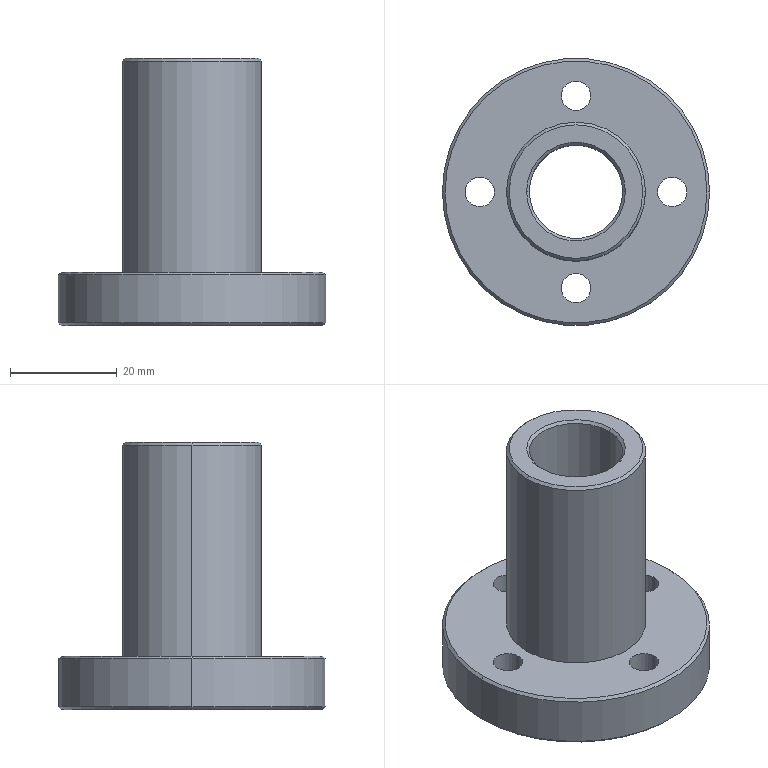Component | SolidWorks | OPW-05-011-1 | 1 solid | 39 faces | box 50 x 50 x 50 mm | volume 26737 mm3 | cylinder 22 | cone 10 | plane 7 | commonest cylinder face diameters 10 x8 5.5 x8 17.5 x2 26 x2 50 x2 | material Brass
STEP:
#1=CARTESIAN_POINT('',(-0.9411,0.4724,-1.575));
#2=VERTEX_POINT('',#1);
#3=CARTESIAN_POINT('',(0.988,0.4724,-1.575));
#4=VERTEX_POINT('',#3);
#5=CARTESIAN_POINT('',(0.02348,0.4724,-1.575));
#6=DIRECTION('',(-0.,-0.,-1.));
#7=DIRECTION('',(-1.,-0.,0.));
#8=AXIS2_PLACEMENT_3D('',#5,#6,#7);
#9=CIRCLE('',#8,0.9646);
#10=EDGE_CURVE('',#2,#4,#9,.T.);
#11=ORIENTED_EDGE('',*,*,#10,.F.);
#12=CARTESIAN_POINT('',(-0.9608,0.4724,-1.555));
#13=VERTEX_POINT('',#12);
#14=CARTESIAN_POINT('',(-0.9411,0.4724,-1.575));
#15=DIRECTION('',(-0.7071,0.,0.7071));
#16=VECTOR('',#15,39.37);
#17=LINE('',#14,#16);
#18=EDGE_CURVE('',#2,#13,#17,.T.);
#19=ORIENTED_EDGE('',*,*,#18,.T.);
#20=CARTESIAN_POINT('',(1.008,0.4724,-1.555));
#21=VERTEX_POINT('',#20);
#22=CARTESIAN_POINT('',(0.02348,0.4724,-1.555));
#23=DIRECTION('',(0.,0.,1.));
#24=DIRECTION('',(-1.,-0.,0.));
#25=AXIS2_PLACEMENT_3D('',#22,#23,#24);
#26=CIRCLE('',#25,0.9843);
#27=EDGE_CURVE('',#21,#13,#26,.T.);
#28=ORIENTED_EDGE('',*,*,#27,.F.);
#29=CARTESIAN_POINT('',(0.988,0.4724,-1.575));
#30=DIRECTION('',(0.7071,0.,0.7071));
#31=VECTOR('',#30,39.37);
#32=LINE('',#29,#31);
#33=EDGE_CURVE('',#4,#21,#32,.T.);
#34=ORIENTED_EDGE('',*,*,#33,.F.);
#35=EDGE_LOOP('',(#11,#19,#28,#34));
#36=FACE_OUTER_BOUND('',#35,.T.);
#37=CARTESIAN_POINT('',(0.02348,0.4724,-1.575));
#38=DIRECTION('',(0.,0.,1.));
#39=DIRECTION('',(1.,0.,0.));
#40=AXIS2_PLACEMENT_3D('',#37,#38,#39);
#41=CONICAL_SURFACE('',#40,0.9646,0.7854);
#42=ADVANCED_FACE('',(#36),#41,.T.);
#43=CARTESIAN_POINT('',(0.988,0.4724,-1.181));
#44=VERTEX_POINT('',#43);
#45=CARTESIAN_POINT('',(-0.9411,0.4724,-1.181));
#46=VERTEX_POINT('',#45);
#47=CARTESIAN_POINT('',(0.02348,0.4724,-1.181));
#48=DIRECTION('',(0.,0.,1.));
#49=DIRECTION('',(1.,0.,-0.));
#50=AXIS2_PLACEMENT_3D('',#47,#48,#49);
#51=CIRCLE('',#50,0.9646);
#52=EDGE_CURVE('',#44,#46,#51,.T.);
#53=ORIENTED_EDGE('',*,*,#52,.F.);
#54=CARTESIAN_POINT('',(1.008,0.4724,-1.201));
#55=VERTEX_POINT('',#54);
#56=CARTESIAN_POINT('',(0.988,0.4724,-1.181));
#57=DIRECTION('',(0.7071,0.,-0.7071));
#58=VECTOR('',#57,39.37);
#59=LINE('',#56,#58);
#60=EDGE_CURVE('',#44,#55,#59,.T.);
#61=ORIENTED_EDGE('',*,*,#60,.T.);
#62=CARTESIAN_POINT('',(-0.9608,0.4724,-1.201));
#63=VERTEX_POINT('',#62);
#64=CARTESIAN_POINT('',(0.02348,0.4724,-1.201));
#65=DIRECTION('',(-0.,-0.,-1.));
#66=DIRECTION('',(1.,0.,-0.));
#67=AXIS2_PLACEMENT_3D('',#64,#65,#66);
#68=CIRCLE('',#67,0.9843);
#69=EDGE_CURVE('',#63,#55,#68,.T.);
#70=ORIENTED_EDGE('',*,*,#69,.F.);
#71=CARTESIAN_POINT('',(-0.9411,0.4724,-1.181));
#72=DIRECTION('',(-0.7071,-0.,-0.7071));
#73=VECTOR('',#72,39.37);
#74=LINE('',#71,#73);
#75=EDGE_CURVE('',#46,#63,#74,.T.);
#76=ORIENTED_EDGE('',*,*,#75,.F.);
#77=EDGE_LOOP('',(#53,#61,#70,#76));
#78=FACE_OUTER_BOUND('',#77,.T.);
#79=CARTESIAN_POINT('',(0.02348,0.4724,-1.181));
#80=DIRECTION('',(-0.,-0.,-1.));
#81=DIRECTION('',(-1.,-0.,0.));
#82=AXIS2_PLACEMENT_3D('',#79,#80,#81);
#83=CONICAL_SURFACE('',#82,0.9646,0.7854);
#84=ADVANCED_FACE('',(#78),#83,.T.);
#85=CARTESIAN_POINT('',(0.368,0.4724,-1.555));
#86=VERTEX_POINT('',#85);
#87=CARTESIAN_POINT('',(-0.321,0.4724,-1.555));
#88=VERTEX_POINT('',#87);
#89=CARTESIAN_POINT('',(0.02348,0.4724,-1.555));
#90=DIRECTION('',(-0.,-0.,-1.));
#91=DIRECTION('',(-1.,0.,0.));
#92=AXIS2_PLACEMENT_3D('',#89,#90,#91);
#93=CIRCLE('',#92,0.3445);
#94=EDGE_CURVE('',#86,#88,#93,.T.);
#95=ORIENTED_EDGE('',*,*,#94,.F.);
#96=CARTESIAN_POINT('',(0.3877,0.4724,-1.575));
#97=VERTEX_POINT('',#96);
#98=CARTESIAN_POINT('',(0.368,0.4724,-1.555));
#99=DIRECTION('',(0.7071,0.,-0.7071));
#100=VECTOR('',#99,39.37);
#101=LINE('',#98,#100);
#102=EDGE_CURVE('',#86,#97,#101,.T.);
#103=ORIENTED_EDGE('',*,*,#102,.T.);
#104=CARTESIAN_POINT('',(-0.3407,0.4724,-1.575));
#105=VERTEX_POINT('',#104);
#106=CARTESIAN_POINT('',(0.02348,0.4724,-1.575));
#107=DIRECTION('',(0.,0.,1.));
#108=DIRECTION('',(-1.,0.,0.));
#109=AXIS2_PLACEMENT_3D('',#106,#107,#108);
#110=CIRCLE('',#109,0.3642);
#111=EDGE_CURVE('',#105,#97,#110,.T.);
#112=ORIENTED_EDGE('',*,*,#111,.F.);
#113=CARTESIAN_POINT('',(-0.321,0.4724,-1.555));
#114=DIRECTION('',(-0.7071,-0.,-0.7071));
#115=VECTOR('',#114,39.37);
#116=LINE('',#113,#115);
#117=EDGE_CURVE('',#88,#105,#116,.T.);
#118=ORIENTED_EDGE('',*,*,#117,.F.);
#119=EDGE_LOOP('',(#95,#103,#112,#118));
#120=FACE_OUTER_BOUND('',#119,.T.);
#121=CARTESIAN_POINT('',(0.02348,0.4724,-1.555));
#122=DIRECTION('',(-0.,-0.,-1.));
#123=DIRECTION('',(-1.,0.,0.));
#124=AXIS2_PLACEMENT_3D('',#121,#122,#123);
#125=CONICAL_SURFACE('',#124,0.3445,0.7854);
#126=ADVANCED_FACE('',(#120),#125,.F.);
#127=CARTESIAN_POINT('',(-0.321,0.4724,0.374));
#128=VERTEX_POINT('',#127);
#129=CARTESIAN_POINT('',(0.368,0.4724,0.374));
#130=VERTEX_POINT('',#129);
#131=CARTESIAN_POINT('',(0.02348,0.4724,0.374));
#132=DIRECTION('',(0.,0.,1.));
#133=DIRECTION('',(-1.,0.,0.));
#134=AXIS2_PLACEMENT_3D('',#131,#132,#133);
#135=CIRCLE('',#134,0.3445);
#136=EDGE_CURVE('',#128,#130,#135,.T.);
#137=ORIENTED_EDGE('',*,*,#136,.F.);
#138=CARTESIAN_POINT('',(-0.3407,0.4724,0.3937));
#139=VERTEX_POINT('',#138);
#140=CARTESIAN_POINT('',(-0.3407,0.4724,0.3937));
#141=DIRECTION('',(-0.7071,0.,0.7071));
#142=VECTOR('',#141,39.37);
#143=LINE('',#140,#142);
#144=EDGE_CURVE('',#128,#139,#143,.T.);
#145=ORIENTED_EDGE('',*,*,#144,.T.);
#146=CARTESIAN_POINT('',(0.3877,0.4724,0.3937));
#147=VERTEX_POINT('',#146);
#148=CARTESIAN_POINT('',(0.02348,0.4724,0.3937));
#149=DIRECTION('',(-0.,-0.,-1.));
#150=DIRECTION('',(-1.,0.,0.));
#151=AXIS2_PLACEMENT_3D('',#148,#149,#150);
#152=CIRCLE('',#151,0.3642);
#153=EDGE_CURVE('',#147,#139,#152,.T.);
#154=ORIENTED_EDGE('',*,*,#153,.F.);
#155=CARTESIAN_POINT('',(0.3877,0.4724,0.3937));
#156=DIRECTION('',(0.7071,0.,0.7071));
#157=VECTOR('',#156,39.37);
#158=LINE('',#155,#157);
#159=EDGE_CURVE('',#130,#147,#158,.T.);
#160=ORIENTED_EDGE('',*,*,#159,.F.);
#161=EDGE_LOOP('',(#137,#145,#154,#160));
#162=FACE_OUTER_BOUND('',#161,.T.);
#163=CARTESIAN_POINT('',(0.02348,0.4724,0.3937));
#164=DIRECTION('',(0.,0.,1.));
#165=DIRECTION('',(1.,0.,-0.));
#166=AXIS2_PLACEMENT_3D('',#163,#164,#165);
#167=CONICAL_SURFACE('',#166,0.3642,0.7854);
#168=ADVANCED_FACE('',(#162),#167,.F.);
#169=CARTESIAN_POINT('',(0.5156,0.4724,0.3937));
#170=VERTEX_POINT('',#169);
#171=CARTESIAN_POINT('',(-0.4686,0.4724,0.3937));
#172=VERTEX_POINT('',#171);
#173=CARTESIAN_POINT('',(0.02348,0.4724,0.3937));
#174=DIRECTION('',(0.,0.,1.));
#175=DIRECTION('',(-1.,0.,0.));
#176=AXIS2_PLACEMENT_3D('',#173,#174,#175);
#177=CIRCLE('',#176,0.4921);
#178=EDGE_CURVE('',#170,#172,#177,.T.);
#179=ORIENTED_EDGE('',*,*,#178,.F.);
#180=CARTESIAN_POINT('',(0.5353,0.4724,0.374));
#181=VERTEX_POINT('',#180);
#182=CARTESIAN_POINT('',(0.5156,0.4724,0.3937));
#183=DIRECTION('',(0.7071,0.,-0.7071));
#184=VECTOR('',#183,39.37);
#185=LINE('',#182,#184);
#186=EDGE_CURVE('',#170,#181,#185,.T.);
#187=ORIENTED_EDGE('',*,*,#186,.T.);
#188=CARTESIAN_POINT('',(-0.4883,0.4724,0.374));
#189=VERTEX_POINT('',#188);
#190=CARTESIAN_POINT('',(0.02348,0.4724,0.374));
#191=DIRECTION('',(-0.,-0.,-1.));
#192=DIRECTION('',(-1.,0.,0.));
#193=AXIS2_PLACEMENT_3D('',#190,#191,#192);
#194=CIRCLE('',#193,0.5118);
#195=EDGE_CURVE('',#189,#181,#194,.T.);
#196=ORIENTED_EDGE('',*,*,#195,.F.);
#197=CARTESIAN_POINT('',(-0.4686,0.4724,0.3937));
#198=DIRECTION('',(-0.7071,-0.,-0.7071));
#199=VECTOR('',#198,39.37);
#200=LINE('',#197,#199);
#201=EDGE_CURVE('',#172,#189,#200,.T.);
#202=ORIENTED_EDGE('',*,*,#201,.F.);
#203=EDGE_LOOP('',(#179,#187,#196,#202));
#204=FACE_OUTER_BOUND('',#203,.T.);
#205=CARTESIAN_POINT('',(0.02348,0.4724,0.3937));
#206=DIRECTION('',(-0.,-0.,-1.));
#207=DIRECTION('',(-1.,0.,0.));
#208=AXIS2_PLACEMENT_3D('',#205,#206,#207);
#209=CONICAL_SURFACE('',#208,0.4921,0.7854);
#210=ADVANCED_FACE('',(#204),#209,.T.);
#211=CARTESIAN_POINT('',(0.929,0.4724,-1.378));
#212=VERTEX_POINT('',#211);
#213=CARTESIAN_POINT('',(0.5353,0.4724,-1.378));
#214=VERTEX_POINT('',#213);
#215=CARTESIAN_POINT('',(0.7321,0.4724,-1.378));
#216=DIRECTION('',(-0.,-0.,-1.));
#217=DIRECTION('',(-1.,0.,0.));
#218=AXIS2_PLACEMENT_3D('',#215,#216,#217);
#219=CIRCLE('',#218,0.1969);
#220=EDGE_CURVE('',#212,#214,#219,.T.);
#221=ORIENTED_EDGE('',*,*,#220,.F.);
#222=CARTESIAN_POINT('',(0.929,0.4724,-1.575));
#223=VERTEX_POINT('',#222);
#224=CARTESIAN_POINT('',(0.929,0.4724,-1.575));
#225=DIRECTION('',(-0.,-0.,-1.));
#226=VECTOR('',#225,39.37);
#227=LINE('',#224,#226);
#228=EDGE_CURVE('',#212,#223,#227,.T.);
#229=ORIENTED_EDGE('',*,*,#228,.T.);
#230=CARTESIAN_POINT('',(0.5353,0.4724,-1.575));
#231=VERTEX_POINT('',#230);
#232=CARTESIAN_POINT('',(0.7321,0.4724,-1.575));
#233=DIRECTION('',(-0.,-0.,-1.));
#234=DIRECTION('',(-1.,0.,0.));
#235=AXIS2_PLACEMENT_3D('',#232,#233,#234);
#236=CIRCLE('',#235,0.1969);
#237=EDGE_CURVE('',#223,#231,#236,.T.);
#238=ORIENTED_EDGE('',*,*,#237,.T.);
#239=CARTESIAN_POINT('',(0.5353,0.4724,-1.575));
#240=DIRECTION('',(-0.,-0.,-1.));
#241=VECTOR('',#240,39.37);
#242=LINE('',#239,#241);
#243=EDGE_CURVE('',#214,#231,#242,.T.);
#244=ORIENTED_EDGE('',*,*,#243,.F.);
#245=EDGE_LOOP('',(#221,#229,#238,#244));
#246=FACE_OUTER_BOUND('',#245,.T.);
#247=CARTESIAN_POINT('',(0.7321,0.4724,-1.575));
#248=DIRECTION('',(-0.,-0.,-1.));
#249=DIRECTION('',(-1.,0.,0.));
#250=AXIS2_PLACEMENT_3D('',#247,#248,#249);
#251=CYLINDRICAL_SURFACE('',#250,0.1969);
#252=ADVANCED_FACE('',(#246),#251,.F.);
#253=CARTESIAN_POINT('',(0.6239,0.4724,-1.181));
#254=VERTEX_POINT('',#253);
#255=CARTESIAN_POINT('',(0.8404,0.4724,-1.181));
#256=VERTEX_POINT('',#255);
#257=CARTESIAN_POINT('',(0.7321,0.4724,-1.181));
#258=DIRECTION('',(0.,0.,1.));
#259=DIRECTION('',(1.,0.,0.));
#260=AXIS2_PLACEMENT_3D('',#257,#258,#259);
#261=CIRCLE('',#260,0.1083);
#262=EDGE_CURVE('',#254,#256,#261,.T.);
#263=ORIENTED_EDGE('',*,*,#262,.T.);
#264=CARTESIAN_POINT('',(0.8404,0.4724,-1.378));
#265=VERTEX_POINT('',#264);
#266=CARTESIAN_POINT('',(0.8404,0.4724,-1.575));
#267=DIRECTION('',(-0.,-0.,-1.));
#268=VECTOR('',#267,39.37);
#269=LINE('',#266,#268);
#270=EDGE_CURVE('',#256,#265,#269,.T.);
#271=ORIENTED_EDGE('',*,*,#270,.T.);
#272=CARTESIAN_POINT('',(0.6239,0.4724,-1.378));
#273=VERTEX_POINT('',#272);
#274=CARTESIAN_POINT('',(0.7321,0.4724,-1.378));
#275=DIRECTION('',(-0.,-0.,-1.));
#276=DIRECTION('',(-1.,0.,0.));
#277=AXIS2_PLACEMENT_3D('',#274,#275,#276);
#278=CIRCLE('',#277,0.1083);
#279=EDGE_CURVE('',#265,#273,#278,.T.);
#280=ORIENTED_EDGE('',*,*,#279,.T.);
#281=CARTESIAN_POINT('',(0.6239,0.4724,-1.575));
#282=DIRECTION('',(-0.,-0.,-1.));
#283=VECTOR('',#282,39.37);
#284=LINE('',#281,#283);
#285=EDGE_CURVE('',#254,#273,#284,.T.);
#286=ORIENTED_EDGE('',*,*,#285,.F.);
#287=EDGE_LOOP('',(#263,#271,#280,#286));
#288=FACE_OUTER_BOUND('',#287,.T.);
#289=CARTESIAN_POINT('',(0.7321,0.4724,-1.575));
#290=DIRECTION('',(-0.,-0.,-1.));
#291=DIRECTION('',(-1.,0.,0.));
#292=AXIS2_PLACEMENT_3D('',#289,#290,#291);
#293=CYLINDRICAL_SURFACE('',#292,0.1083);
#294=ADVANCED_FACE('',(#288),#293,.F.);
#295=CARTESIAN_POINT('',(0.2203,-0.2363,-1.378));
#296=VERTEX_POINT('',#295);
#297=CARTESIAN_POINT('',(-0.1734,-0.2363,-1.378));
#298=VERTEX_POINT('',#297);
#299=CARTESIAN_POINT('',(0.02348,-0.2363,-1.378));
#300=DIRECTION('',(-0.,-0.,-1.));
#301=DIRECTION('',(-1.,0.,0.));
#302=AXIS2_PLACEMENT_3D('',#299,#300,#301);
#303=CIRCLE('',#302,0.1969);
#304=EDGE_CURVE('',#296,#298,#303,.T.);
#305=ORIENTED_EDGE('',*,*,#304,.F.);
#306=CARTESIAN_POINT('',(0.2203,-0.2363,-1.575));
#307=VERTEX_POINT('',#306);
#308=CARTESIAN_POINT('',(0.2203,-0.2363,-1.575));
#309=DIRECTION('',(-0.,-0.,-1.));
#310=VECTOR('',#309,39.37);
#311=LINE('',#308,#310);
#312=EDGE_CURVE('',#296,#307,#311,.T.);
#313=ORIENTED_EDGE('',*,*,#312,.T.);
#314=CARTESIAN_POINT('',(-0.1734,-0.2363,-1.575));
#315=VERTEX_POINT('',#314);
#316=CARTESIAN_POINT('',(0.02348,-0.2363,-1.575));
#317=DIRECTION('',(-0.,-0.,-1.));
#318=DIRECTION('',(-1.,0.,0.));
#319=AXIS2_PLACEMENT_3D('',#316,#317,#318);
#320=CIRCLE('',#319,0.1969);
#321=EDGE_CURVE('',#307,#315,#320,.T.);
#322=ORIENTED_EDGE('',*,*,#321,.T.);
#323=CARTESIAN_POINT('',(-0.1734,-0.2363,-1.575));
#324=DIRECTION('',(-0.,-0.,-1.));
#325=VECTOR('',#324,39.37);
#326=LINE('',#323,#325);
#327=EDGE_CURVE('',#298,#315,#326,.T.);
#328=ORIENTED_EDGE('',*,*,#327,.F.);
#329=EDGE_LOOP('',(#305,#313,#322,#328));
#330=FACE_OUTER_BOUND('',#329,.T.);
#331=CARTESIAN_POINT('',(0.02348,-0.2363,-1.575));
#332=DIRECTION('',(-0.,-0.,-1.));
#333=DIRECTION('',(-1.,0.,0.));
#334=AXIS2_PLACEMENT_3D('',#331,#332,#333);
#335=CYLINDRICAL_SURFACE('',#334,0.1969);
#336=ADVANCED_FACE('',(#330),#335,.F.);
#337=CARTESIAN_POINT('',(-0.08478,-0.2363,-1.181));
#338=VERTEX_POINT('',#337);
#339=CARTESIAN_POINT('',(0.1318,-0.2363,-1.181));
#340=VERTEX_POINT('',#339);
#341=CARTESIAN_POINT('',(0.02348,-0.2363,-1.181));
#342=DIRECTION('',(0.,0.,1.));
#343=DIRECTION('',(1.,0.,0.));
#344=AXIS2_PLACEMENT_3D('',#341,#342,#343);
#345=CIRCLE('',#344,0.1083);
#346=EDGE_CURVE('',#338,#340,#345,.T.);
#347=ORIENTED_EDGE('',*,*,#346,.T.);
#348=CARTESIAN_POINT('',(0.1318,-0.2363,-1.378));
#349=VERTEX_POINT('',#348);
#350=CARTESIAN_POINT('',(0.1318,-0.2363,-1.575));
#351=DIRECTION('',(-0.,-0.,-1.));
#352=VECTOR('',#351,39.37);
#353=LINE('',#350,#352);
#354=EDGE_CURVE('',#340,#349,#353,.T.);
#355=ORIENTED_EDGE('',*,*,#354,.T.);
#356=CARTESIAN_POINT('',(-0.08478,-0.2363,-1.378));
#357=VERTEX_POINT('',#356);
#358=CARTESIAN_POINT('',(0.02348,-0.2363,-1.378));
#359=DIRECTION('',(-0.,-0.,-1.));
#360=DIRECTION('',(-1.,0.,0.));
#361=AXIS2_PLACEMENT_3D('',#358,#359,#360);
#362=CIRCLE('',#361,0.1083);
#363=EDGE_CURVE('',#349,#357,#362,.T.);
#364=ORIENTED_EDGE('',*,*,#363,.T.);
#365=CARTESIAN_POINT('',(-0.08478,-0.2363,-1.575));
#366=DIRECTION('',(-0.,-0.,-1.));
#367=VECTOR('',#366,39.37);
#368=LINE('',#365,#367);
#369=EDGE_CURVE('',#338,#357,#368,.T.);
#370=ORIENTED_EDGE('',*,*,#369,.F.);
#371=EDGE_LOOP('',(#347,#355,#364,#370));
#372=FACE_OUTER_BOUND('',#371,.T.);
#373=CARTESIAN_POINT('',(0.02348,-0.2363,-1.575));
#374=DIRECTION('',(-0.,-0.,-1.));
#375=DIRECTION('',(-1.,0.,0.));
#376=AXIS2_PLACEMENT_3D('',#373,#374,#375);
#377=CYLINDRICAL_SURFACE('',#376,0.1083);
#378=ADVANCED_FACE('',(#372),#377,.F.);
#379=CARTESIAN_POINT('',(-0.4883,0.4724,-1.378));
#380=VERTEX_POINT('',#379);
#381=CARTESIAN_POINT('',(-0.882,0.4724,-1.378));
#382=VERTEX_POINT('',#381);
#383=CARTESIAN_POINT('',(-0.6852,0.4724,-1.378));
#384=DIRECTION('',(-0.,-0.,-1.));
#385=DIRECTION('',(-1.,0.,0.));
#386=AXIS2_PLACEMENT_3D('',#383,#384,#385);
#387=CIRCLE('',#386,0.1969);
#388=EDGE_CURVE('',#380,#382,#387,.T.);
#389=ORIENTED_EDGE('',*,*,#388,.F.);
#390=CARTESIAN_POINT('',(-0.4883,0.4724,-1.575));
#391=VERTEX_POINT('',#390);
#392=CARTESIAN_POINT('',(-0.4883,0.4724,-1.575));
#393=DIRECTION('',(-0.,-0.,-1.));
#394=VECTOR('',#393,39.37);
#395=LINE('',#392,#394);
#396=EDGE_CURVE('',#380,#391,#395,.T.);
#397=ORIENTED_EDGE('',*,*,#396,.T.);
#398=CARTESIAN_POINT('',(-0.882,0.4724,-1.575));
#399=VERTEX_POINT('',#398);
#400=CARTESIAN_POINT('',(-0.6852,0.4724,-1.575));
#401=DIRECTION('',(-0.,-0.,-1.));
#402=DIRECTION('',(-1.,0.,0.));
#403=AXIS2_PLACEMENT_3D('',#400,#401,#402);
#404=CIRCLE('',#403,0.1969);
#405=EDGE_CURVE('',#391,#399,#404,.T.);
#406=ORIENTED_EDGE('',*,*,#405,.T.);
#407=CARTESIAN_POINT('',(-0.882,0.4724,-1.575));
#408=DIRECTION('',(-0.,-0.,-1.));
#409=VECTOR('',#408,39.37);
#410=LINE('',#407,#409);
#411=EDGE_CURVE('',#382,#399,#410,.T.);
#412=ORIENTED_EDGE('',*,*,#411,.F.);
#413=EDGE_LOOP('',(#389,#397,#406,#412));
#414=FACE_OUTER_BOUND('',#413,.T.);
#415=CARTESIAN_POINT('',(-0.6852,0.4724,-1.575));
#416=DIRECTION('',(-0.,-0.,-1.));
#417=DIRECTION('',(-1.,0.,0.));
#418=AXIS2_PLACEMENT_3D('',#415,#416,#417);
#419=CYLINDRICAL_SURFACE('',#418,0.1969);
#420=ADVANCED_FACE('',(#414),#419,.F.);
#421=CARTESIAN_POINT('',(-0.7934,0.4724,-1.181));
#422=VERTEX_POINT('',#421);
#423=CARTESIAN_POINT('',(-0.5769,0.4724,-1.181));
#424=VERTEX_POINT('',#423);
#425=CARTESIAN_POINT('',(-0.6852,0.4724,-1.181));
#426=DIRECTION('',(0.,0.,1.));
#427=DIRECTION('',(1.,0.,0.));
#428=AXIS2_PLACEMENT_3D('',#425,#426,#427);
#429=CIRCLE('',#428,0.1083);
#430=EDGE_CURVE('',#422,#424,#429,.T.);
#431=ORIENTED_EDGE('',*,*,#430,.T.);
#432=CARTESIAN_POINT('',(-0.5769,0.4724,-1.378));
#433=VERTEX_POINT('',#432);
#434=CARTESIAN_POINT('',(-0.5769,0.4724,-1.575));
#435=DIRECTION('',(-0.,-0.,-1.));
#436=VECTOR('',#435,39.37);
#437=LINE('',#434,#436);
#438=EDGE_CURVE('',#424,#433,#437,.T.);
#439=ORIENTED_EDGE('',*,*,#438,.T.);
#440=CARTESIAN_POINT('',(-0.7934,0.4724,-1.378));
#441=VERTEX_POINT('',#440);
#442=CARTESIAN_POINT('',(-0.6852,0.4724,-1.378));
#443=DIRECTION('',(-0.,-0.,-1.));
#444=DIRECTION('',(-1.,0.,0.));
#445=AXIS2_PLACEMENT_3D('',#442,#443,#444);
#446=CIRCLE('',#445,0.1083);
#447=EDGE_CURVE('',#433,#441,#446,.T.);
#448=ORIENTED_EDGE('',*,*,#447,.T.);
#449=CARTESIAN_POINT('',(-0.7934,0.4724,-1.575));
#450=DIRECTION('',(-0.,-0.,-1.));
#451=VECTOR('',#450,39.37);
#452=LINE('',#449,#451);
#453=EDGE_CURVE('',#422,#441,#452,.T.);
#454=ORIENTED_EDGE('',*,*,#453,.F.);
#455=EDGE_LOOP('',(#431,#439,#448,#454));
#456=FACE_OUTER_BOUND('',#455,.T.);
#457=CARTESIAN_POINT('',(-0.6852,0.4724,-1.575));
#458=DIRECTION('',(-0.,-0.,-1.));
#459=DIRECTION('',(-1.,0.,0.));
#460=AXIS2_PLACEMENT_3D('',#457,#458,#459);
#461=CYLINDRICAL_SURFACE('',#460,0.1083);
#462=ADVANCED_FACE('',(#456),#461,.F.);
#463=CARTESIAN_POINT('',(0.2203,1.181,-1.378));
#464=VERTEX_POINT('',#463);
#465=CARTESIAN_POINT('',(-0.1734,1.181,-1.378));
#466=VERTEX_POINT('',#465);
#467=CARTESIAN_POINT('',(0.02348,1.181,-1.378));
#468=DIRECTION('',(-0.,-0.,-1.));
#469=DIRECTION('',(-1.,0.,0.));
#470=AXIS2_PLACEMENT_3D('',#467,#468,#469);
#471=CIRCLE('',#470,0.1969);
#472=EDGE_CURVE('',#464,#466,#471,.T.);
#473=ORIENTED_EDGE('',*,*,#472,.F.);
#474=CARTESIAN_POINT('',(0.2203,1.181,-1.575));
#475=VERTEX_POINT('',#474);
#476=CARTESIAN_POINT('',(0.2203,1.181,-1.575));
#477=DIRECTION('',(-0.,-0.,-1.));
#478=VECTOR('',#477,39.37);
#479=LINE('',#476,#478);
#480=EDGE_CURVE('',#464,#475,#479,.T.);
#481=ORIENTED_EDGE('',*,*,#480,.T.);
#482=CARTESIAN_POINT('',(-0.1734,1.181,-1.575));
#483=VERTEX_POINT('',#482);
#484=CARTESIAN_POINT('',(0.02348,1.181,-1.575));
#485=DIRECTION('',(-0.,-0.,-1.));
#486=DIRECTION('',(-1.,0.,0.));
#487=AXIS2_PLACEMENT_3D('',#484,#485,#486);
#488=CIRCLE('',#487,0.1969);
#489=EDGE_CURVE('',#475,#483,#488,.T.);
#490=ORIENTED_EDGE('',*,*,#489,.T.);
#491=CARTESIAN_POINT('',(-0.1734,1.181,-1.575));
#492=DIRECTION('',(-0.,-0.,-1.));
#493=VECTOR('',#492,39.37);
#494=LINE('',#491,#493);
#495=EDGE_CURVE('',#466,#483,#494,.T.);
#496=ORIENTED_EDGE('',*,*,#495,.F.);
#497=EDGE_LOOP('',(#473,#481,#490,#496));
#498=FACE_OUTER_BOUND('',#497,.T.);
#499=CARTESIAN_POINT('',(0.02348,1.181,-1.575));
#500=DIRECTION('',(-0.,-0.,-1.));
#501=DIRECTION('',(-1.,0.,0.));
#502=AXIS2_PLACEMENT_3D('',#499,#500,#501);
#503=CYLINDRICAL_SURFACE('',#502,0.1969);
#504=ADVANCED_FACE('',(#498),#503,.F.);
#505=CARTESIAN_POINT('',(-0.08478,1.181,-1.181));
#506=VERTEX_POINT('',#505);
#507=CARTESIAN_POINT('',(0.1318,1.181,-1.181));
#508=VERTEX_POINT('',#507);
#509=CARTESIAN_POINT('',(0.02348,1.181,-1.181));
#510=DIRECTION('',(0.,0.,1.));
#511=DIRECTION('',(1.,0.,0.));
#512=AXIS2_PLACEMENT_3D('',#509,#510,#511);
#513=CIRCLE('',#512,0.1083);
#514=EDGE_CURVE('',#506,#508,#513,.T.);
#515=ORIENTED_EDGE('',*,*,#514,.T.);
#516=CARTESIAN_POINT('',(0.1318,1.181,-1.378));
#517=VERTEX_POINT('',#516);
#518=CARTESIAN_POINT('',(0.1318,1.181,-1.575));
#519=DIRECTION('',(-0.,-0.,-1.));
#520=VECTOR('',#519,39.37);
#521=LINE('',#518,#520);
#522=EDGE_CURVE('',#508,#517,#521,.T.);
#523=ORIENTED_EDGE('',*,*,#522,.T.);
#524=CARTESIAN_POINT('',(-0.08478,1.181,-1.378));
#525=VERTEX_POINT('',#524);
#526=CARTESIAN_POINT('',(0.02348,1.181,-1.378));
#527=DIRECTION('',(-0.,-0.,-1.));
#528=DIRECTION('',(-1.,0.,0.));
#529=AXIS2_PLACEMENT_3D('',#526,#527,#528);
#530=CIRCLE('',#529,0.1083);
#531=EDGE_CURVE('',#517,#525,#530,.T.);
#532=ORIENTED_EDGE('',*,*,#531,.T.);
#533=CARTESIAN_POINT('',(-0.08478,1.181,-1.575));
#534=DIRECTION('',(-0.,-0.,-1.));
#535=VECTOR('',#534,39.37);
#536=LINE('',#533,#535);
#537=EDGE_CURVE('',#506,#525,#536,.T.);
#538=ORIENTED_EDGE('',*,*,#537,.F.);
#539=EDGE_LOOP('',(#515,#523,#532,#538));
#540=FACE_OUTER_BOUND('',#539,.T.);
#541=CARTESIAN_POINT('',(0.02348,1.181,-1.575));
#542=DIRECTION('',(-0.,-0.,-1.));
#543=DIRECTION('',(-1.,0.,0.));
#544=AXIS2_PLACEMENT_3D('',#541,#542,#543);
#545=CYLINDRICAL_SURFACE('',#544,0.1083);
#546=ADVANCED_FACE('',(#540),#545,.F.);
#547=ORIENTED_EDGE('',*,*,#136,.T.);
#548=CARTESIAN_POINT('',(0.368,0.4724,-1.575));
#549=DIRECTION('',(-0.,-0.,-1.));
#550=VECTOR('',#549,39.37);
#551=LINE('',#548,#550);
#552=EDGE_CURVE('',#130,#86,#551,.T.);
#553=ORIENTED_EDGE('',*,*,#552,.T.);
#554=ORIENTED_EDGE('',*,*,#94,.T.);
#555=CARTESIAN_POINT('',(-0.321,0.4724,-1.575));
#556=DIRECTION('',(-0.,-0.,-1.));
#557=VECTOR('',#556,39.37);
#558=LINE('',#555,#557);
#559=EDGE_CURVE('',#128,#88,#558,.T.);
#560=ORIENTED_EDGE('',*,*,#559,.F.);
#561=EDGE_LOOP('',(#547,#553,#554,#560));
#562=FACE_OUTER_BOUND('',#561,.T.);
#563=CARTESIAN_POINT('',(0.02348,0.4724,-1.575));
#564=DIRECTION('',(-0.,-0.,-1.));
#565=DIRECTION('',(-1.,0.,0.));
#566=AXIS2_PLACEMENT_3D('',#563,#564,#565);
#567=CYLINDRICAL_SURFACE('',#566,0.3445);
#568=ADVANCED_FACE('',(#562),#567,.F.);
#569=CARTESIAN_POINT('',(0.5353,0.4724,-1.181));
#570=VERTEX_POINT('',#569);
#571=CARTESIAN_POINT('',(-0.4883,0.4724,-1.181));
#572=VERTEX_POINT('',#571);
#573=CARTESIAN_POINT('',(0.02348,0.4724,-1.181));
#574=DIRECTION('',(0.,0.,1.));
#575=DIRECTION('',(1.,0.,0.));
#576=AXIS2_PLACEMENT_3D('',#573,#574,#575);
#577=CIRCLE('',#576,0.5118);
#578=EDGE_CURVE('',#570,#572,#577,.T.);
#579=ORIENTED_EDGE('',*,*,#578,.T.);
#580=CARTESIAN_POINT('',(-0.4883,0.4724,-1.181));
#581=DIRECTION('',(0.,0.,1.));
#582=VECTOR('',#581,39.37);
#583=LINE('',#580,#582);
#584=EDGE_CURVE('',#572,#189,#583,.T.);
#585=ORIENTED_EDGE('',*,*,#584,.T.);
#586=ORIENTED_EDGE('',*,*,#195,.T.);
#587=CARTESIAN_POINT('',(0.5353,0.4724,-1.181));
#588=DIRECTION('',(0.,0.,1.));
#589=VECTOR('',#588,39.37);
#590=LINE('',#587,#589);
#591=EDGE_CURVE('',#570,#181,#590,.T.);
#592=ORIENTED_EDGE('',*,*,#591,.F.);
#593=EDGE_LOOP('',(#579,#585,#586,#592));
#594=FACE_OUTER_BOUND('',#593,.T.);
#595=CARTESIAN_POINT('',(0.02348,0.4724,-1.181));
#596=DIRECTION('',(0.,0.,1.));
#597=DIRECTION('',(1.,0.,0.));
#598=AXIS2_PLACEMENT_3D('',#595,#596,#597);
#599=CYLINDRICAL_SURFACE('',#598,0.5118);
#600=ADVANCED_FACE('',(#594),#599,.T.);
#601=ORIENTED_EDGE('',*,*,#27,.T.);
#602=CARTESIAN_POINT('',(-0.9608,0.4724,-1.575));
#603=DIRECTION('',(0.,0.,1.));
#604=VECTOR('',#603,39.37);
#605=LINE('',#602,#604);
#606=EDGE_CURVE('',#13,#63,#605,.T.);
#607=ORIENTED_EDGE('',*,*,#606,.T.);
#608=ORIENTED_EDGE('',*,*,#69,.T.);
#609=CARTESIAN_POINT('',(1.008,0.4724,-1.575));
#610=DIRECTION('',(0.,0.,1.));
#611=VECTOR('',#610,39.37);
#612=LINE('',#609,#611);
#613=EDGE_CURVE('',#21,#55,#612,.T.);
#614=ORIENTED_EDGE('',*,*,#613,.F.);
#615=EDGE_LOOP('',(#601,#607,#608,#614));
#616=FACE_OUTER_BOUND('',#615,.T.);
#617=CARTESIAN_POINT('',(0.02348,0.4724,-1.575));
#618=DIRECTION('',(0.,0.,1.));
#619=DIRECTION('',(1.,0.,0.));
#620=AXIS2_PLACEMENT_3D('',#617,#618,#619);
#621=CYLINDRICAL_SURFACE('',#620,0.9843);
#622=ADVANCED_FACE('',(#616),#621,.T.);
#623=ORIENTED_EDGE('',*,*,#606,.F.);
#624=CARTESIAN_POINT('',(0.02348,0.4724,-1.555));
#625=DIRECTION('',(0.,0.,1.));
#626=DIRECTION('',(-1.,-0.,0.));
#627=AXIS2_PLACEMENT_3D('',#624,#625,#626);
#628=CIRCLE('',#627,0.9843);
#629=EDGE_CURVE('',#13,#21,#628,.T.);
#630=ORIENTED_EDGE('',*,*,#629,.T.);
#631=ORIENTED_EDGE('',*,*,#613,.T.);
#632=CARTESIAN_POINT('',(0.02348,0.4724,-1.201));
#633=DIRECTION('',(-0.,-0.,-1.));
#634=DIRECTION('',(1.,0.,-0.));
#635=AXIS2_PLACEMENT_3D('',#632,#633,#634);
#636=CIRCLE('',#635,0.9843);
#637=EDGE_CURVE('',#55,#63,#636,.T.);
#638=ORIENTED_EDGE('',*,*,#637,.T.);
#639=EDGE_LOOP('',(#623,#630,#631,#638));
#640=FACE_OUTER_BOUND('',#639,.T.);
#641=CARTESIAN_POINT('',(0.02348,0.4724,-1.575));
#642=DIRECTION('',(0.,0.,1.));
#643=DIRECTION('',(1.,0.,0.));
#644=AXIS2_PLACEMENT_3D('',#641,#642,#643);
#645=CYLINDRICAL_SURFACE('',#644,0.9843);
#646=ADVANCED_FACE('',(#640),#645,.T.);
#647=CARTESIAN_POINT('',(0.02348,0.4724,-1.575));
#648=DIRECTION('',(-0.,-0.,-1.));
#649=DIRECTION('',(-1.,-0.,0.));
#650=AXIS2_PLACEMENT_3D('',#647,#648,#649);
#651=CIRCLE('',#650,0.9646);
#652=EDGE_CURVE('',#4,#2,#651,.T.);
#653=ORIENTED_EDGE('',*,*,#652,.T.);
#654=ORIENTED_EDGE('',*,*,#10,.T.);
#655=EDGE_LOOP('',(#653,#654));
#656=FACE_OUTER_BOUND('',#655,.T.);
#657=ORIENTED_EDGE('',*,*,#111,.T.);
#658=CARTESIAN_POINT('',(0.02348,0.4724,-1.575));
#659=DIRECTION('',(0.,0.,1.));
#660=DIRECTION('',(-1.,0.,0.));
#661=AXIS2_PLACEMENT_3D('',#658,#659,#660);
#662=CIRCLE('',#661,0.3642);
#663=EDGE_CURVE('',#97,#105,#662,.T.);
#664=ORIENTED_EDGE('',*,*,#663,.T.);
#665=EDGE_LOOP('',(#657,#664));
#666=FACE_BOUND('',#665,.T.);
#667=CARTESIAN_POINT('',(0.7321,0.4724,-1.575));
#668=DIRECTION('',(-0.,-0.,-1.));
#669=DIRECTION('',(-1.,0.,0.));
#670=AXIS2_PLACEMENT_3D('',#667,#668,#669);
#671=CIRCLE('',#670,0.1969);
#672=EDGE_CURVE('',#231,#223,#671,.T.);
#673=ORIENTED_EDGE('',*,*,#672,.F.);
#674=ORIENTED_EDGE('',*,*,#237,.F.);
#675=EDGE_LOOP('',(#673,#674));
#676=FACE_BOUND('',#675,.T.);
#677=CARTESIAN_POINT('',(0.02348,-0.2363,-1.575));
#678=DIRECTION('',(-0.,-0.,-1.));
#679=DIRECTION('',(-1.,0.,0.));
#680=AXIS2_PLACEMENT_3D('',#677,#678,#679);
#681=CIRCLE('',#680,0.1969);
#682=EDGE_CURVE('',#315,#307,#681,.T.);
#683=ORIENTED_EDGE('',*,*,#682,.F.);
#684=ORIENTED_EDGE('',*,*,#321,.F.);
#685=EDGE_LOOP('',(#683,#684));
#686=FACE_BOUND('',#685,.T.);
#687=CARTESIAN_POINT('',(-0.6852,0.4724,-1.575));
#688=DIRECTION('',(-0.,-0.,-1.));
#689=DIRECTION('',(-1.,0.,0.));
#690=AXIS2_PLACEMENT_3D('',#687,#688,#689);
#691=CIRCLE('',#690,0.1969);
#692=EDGE_CURVE('',#399,#391,#691,.T.);
#693=ORIENTED_EDGE('',*,*,#692,.F.);
#694=ORIENTED_EDGE('',*,*,#405,.F.);
#695=EDGE_LOOP('',(#693,#694));
#696=FACE_BOUND('',#695,.T.);
#697=CARTESIAN_POINT('',(0.02348,1.181,-1.575));
#698=DIRECTION('',(-0.,-0.,-1.));
#699=DIRECTION('',(-1.,0.,0.));
#700=AXIS2_PLACEMENT_3D('',#697,#698,#699);
#701=CIRCLE('',#700,0.1969);
#702=EDGE_CURVE('',#483,#475,#701,.T.);
#703=ORIENTED_EDGE('',*,*,#702,.F.);
#704=ORIENTED_EDGE('',*,*,#489,.F.);
#705=EDGE_LOOP('',(#703,#704));
#706=FACE_BOUND('',#705,.T.);
#707=CARTESIAN_POINT('',(0.02348,0.4724,-1.575));
#708=DIRECTION('',(-0.,-0.,-1.));
#709=DIRECTION('',(-1.,-0.,0.));
#710=AXIS2_PLACEMENT_3D('',#707,#708,#709);
#711=PLANE('',#710);
#712=ADVANCED_FACE('',(#656,#666,#676,#686,#696,#706),#711,.T.);
#713=CARTESIAN_POINT('',(0.02348,0.4724,-1.181));
#714=DIRECTION('',(0.,0.,1.));
#715=DIRECTION('',(1.,0.,-0.));
#716=AXIS2_PLACEMENT_3D('',#713,#714,#715);
#717=CIRCLE('',#716,0.9646);
#718=EDGE_CURVE('',#46,#44,#717,.T.);
#719=ORIENTED_EDGE('',*,*,#718,.T.);
#720=ORIENTED_EDGE('',*,*,#52,.T.);
#721=EDGE_LOOP('',(#719,#720));
#722=FACE_OUTER_BOUND('',#721,.T.);
#723=ORIENTED_EDGE('',*,*,#262,.F.);
#724=CARTESIAN_POINT('',(0.7321,0.4724,-1.181));
#725=DIRECTION('',(0.,0.,1.));
#726=DIRECTION('',(1.,0.,0.));
#727=AXIS2_PLACEMENT_3D('',#724,#725,#726);
#728=CIRCLE('',#727,0.1083);
#729=EDGE_CURVE('',#256,#254,#728,.T.);
#730=ORIENTED_EDGE('',*,*,#729,.F.);
#731=EDGE_LOOP('',(#723,#730));
#732=FACE_BOUND('',#731,.T.);
#733=ORIENTED_EDGE('',*,*,#346,.F.);
#734=CARTESIAN_POINT('',(0.02348,-0.2363,-1.181));
#735=DIRECTION('',(0.,0.,1.));
#736=DIRECTION('',(1.,0.,0.));
#737=AXIS2_PLACEMENT_3D('',#734,#735,#736);
#738=CIRCLE('',#737,0.1083);
#739=EDGE_CURVE('',#340,#338,#738,.T.);
#740=ORIENTED_EDGE('',*,*,#739,.F.);
#741=EDGE_LOOP('',(#733,#740));
#742=FACE_BOUND('',#741,.T.);
#743=ORIENTED_EDGE('',*,*,#430,.F.);
#744=CARTESIAN_POINT('',(-0.6852,0.4724,-1.181));
#745=DIRECTION('',(0.,0.,1.));
#746=DIRECTION('',(1.,0.,0.));
#747=AXIS2_PLACEMENT_3D('',#744,#745,#746);
#748=CIRCLE('',#747,0.1083);
#749=EDGE_CURVE('',#424,#422,#748,.T.);
#750=ORIENTED_EDGE('',*,*,#749,.F.);
#751=EDGE_LOOP('',(#743,#750));
#752=FACE_BOUND('',#751,.T.);
#753=ORIENTED_EDGE('',*,*,#514,.F.);
#754=CARTESIAN_POINT('',(0.02348,1.181,-1.181));
#755=DIRECTION('',(0.,0.,1.));
#756=DIRECTION('',(1.,0.,0.));
#757=AXIS2_PLACEMENT_3D('',#754,#755,#756);
#758=CIRCLE('',#757,0.1083);
#759=EDGE_CURVE('',#508,#506,#758,.T.);
#760=ORIENTED_EDGE('',*,*,#759,.F.);
#761=EDGE_LOOP('',(#753,#760));
#762=FACE_BOUND('',#761,.T.);
#763=ORIENTED_EDGE('',*,*,#578,.F.);
#764=CARTESIAN_POINT('',(0.02348,0.4724,-1.181));
#765=DIRECTION('',(0.,0.,1.));
#766=DIRECTION('',(1.,0.,0.));
#767=AXIS2_PLACEMENT_3D('',#764,#765,#766);
#768=CIRCLE('',#767,0.5118);
#769=EDGE_CURVE('',#572,#570,#768,.T.);
#770=ORIENTED_EDGE('',*,*,#769,.F.);
#771=EDGE_LOOP('',(#763,#770));
#772=FACE_BOUND('',#771,.T.);
#773=CARTESIAN_POINT('',(0.02348,0.4724,-1.181));
#774=DIRECTION('',(0.,0.,1.));
#775=DIRECTION('',(1.,0.,-0.));
#776=AXIS2_PLACEMENT_3D('',#773,#774,#775);
#777=PLANE('',#776);
#778=ADVANCED_FACE('',(#722,#732,#742,#752,#762,#772),#777,.T.);
#779=ORIENTED_EDGE('',*,*,#584,.F.);
#780=ORIENTED_EDGE('',*,*,#769,.T.);
#781=ORIENTED_EDGE('',*,*,#591,.T.);
#782=CARTESIAN_POINT('',(0.02348,0.4724,0.374));
#783=DIRECTION('',(-0.,-0.,-1.));
#784=DIRECTION('',(-1.,0.,0.));
#785=AXIS2_PLACEMENT_3D('',#782,#783,#784);
#786=CIRCLE('',#785,0.5118);
#787=EDGE_CURVE('',#181,#189,#786,.T.);
#788=ORIENTED_EDGE('',*,*,#787,.T.);
#789=EDGE_LOOP('',(#779,#780,#781,#788));
#790=FACE_OUTER_BOUND('',#789,.T.);
#791=CARTESIAN_POINT('',(0.02348,0.4724,-1.181));
#792=DIRECTION('',(0.,0.,1.));
#793=DIRECTION('',(1.,0.,0.));
#794=AXIS2_PLACEMENT_3D('',#791,#792,#793);
#795=CYLINDRICAL_SURFACE('',#794,0.5118);
#796=ADVANCED_FACE('',(#790),#795,.T.);
#797=CARTESIAN_POINT('',(0.02348,0.4724,0.3937));
#798=DIRECTION('',(0.,0.,1.));
#799=DIRECTION('',(-1.,0.,0.));
#800=AXIS2_PLACEMENT_3D('',#797,#798,#799);
#801=CIRCLE('',#800,0.4921);
#802=EDGE_CURVE('',#172,#170,#801,.T.);
#803=ORIENTED_EDGE('',*,*,#802,.T.);
#804=ORIENTED_EDGE('',*,*,#178,.T.);
#805=EDGE_LOOP('',(#803,#804));
#806=FACE_OUTER_BOUND('',#805,.T.);
#807=ORIENTED_EDGE('',*,*,#153,.T.);
#808=CARTESIAN_POINT('',(0.02348,0.4724,0.3937));
#809=DIRECTION('',(-0.,-0.,-1.));
#810=DIRECTION('',(-1.,0.,0.));
#811=AXIS2_PLACEMENT_3D('',#808,#809,#810);
#812=CIRCLE('',#811,0.3642);
#813=EDGE_CURVE('',#139,#147,#812,.T.);
#814=ORIENTED_EDGE('',*,*,#813,.T.);
#815=EDGE_LOOP('',(#807,#814));
#816=FACE_BOUND('',#815,.T.);
#817=CARTESIAN_POINT('',(0.02348,0.4724,0.3937));
#818=DIRECTION('',(-0.,-0.,-1.));
#819=DIRECTION('',(-1.,-0.,0.));
#820=AXIS2_PLACEMENT_3D('',#817,#818,#819);
#821=PLANE('',#820);
#822=ADVANCED_FACE('',(#806,#816),#821,.F.);
#823=ORIENTED_EDGE('',*,*,#552,.F.);
#824=CARTESIAN_POINT('',(0.02348,0.4724,0.374));
#825=DIRECTION('',(0.,0.,1.));
#826=DIRECTION('',(-1.,0.,0.));
#827=AXIS2_PLACEMENT_3D('',#824,#825,#826);
#828=CIRCLE('',#827,0.3445);
#829=EDGE_CURVE('',#130,#128,#828,.T.);
#830=ORIENTED_EDGE('',*,*,#829,.T.);
#831=ORIENTED_EDGE('',*,*,#559,.T.);
#832=CARTESIAN_POINT('',(0.02348,0.4724,-1.555));
#833=DIRECTION('',(-0.,-0.,-1.));
#834=DIRECTION('',(-1.,0.,0.));
#835=AXIS2_PLACEMENT_3D('',#832,#833,#834);
#836=CIRCLE('',#835,0.3445);
#837=EDGE_CURVE('',#88,#86,#836,.T.);
#838=ORIENTED_EDGE('',*,*,#837,.T.);
#839=EDGE_LOOP('',(#823,#830,#831,#838));
#840=FACE_OUTER_BOUND('',#839,.T.);
#841=CARTESIAN_POINT('',(0.02348,0.4724,-1.575));
#842=DIRECTION('',(-0.,-0.,-1.));
#843=DIRECTION('',(-1.,0.,0.));
#844=AXIS2_PLACEMENT_3D('',#841,#842,#843);
#845=CYLINDRICAL_SURFACE('',#844,0.3445);
#846=ADVANCED_FACE('',(#840),#845,.F.);
#847=ORIENTED_EDGE('',*,*,#522,.F.);
#848=ORIENTED_EDGE('',*,*,#759,.T.);
#849=ORIENTED_EDGE('',*,*,#537,.T.);
#850=CARTESIAN_POINT('',(0.02348,1.181,-1.378));
#851=DIRECTION('',(-0.,-0.,-1.));
#852=DIRECTION('',(-1.,0.,0.));
#853=AXIS2_PLACEMENT_3D('',#850,#851,#852);
#854=CIRCLE('',#853,0.1083);
#855=EDGE_CURVE('',#525,#517,#854,.T.);
#856=ORIENTED_EDGE('',*,*,#855,.T.);
#857=EDGE_LOOP('',(#847,#848,#849,#856));
#858=FACE_OUTER_BOUND('',#857,.T.);
#859=CARTESIAN_POINT('',(0.02348,1.181,-1.575));
#860=DIRECTION('',(-0.,-0.,-1.));
#861=DIRECTION('',(-1.,0.,0.));
#862=AXIS2_PLACEMENT_3D('',#859,#860,#861);
#863=CYLINDRICAL_SURFACE('',#862,0.1083);
#864=ADVANCED_FACE('',(#858),#863,.F.);
#865=ORIENTED_EDGE('',*,*,#855,.F.);
#866=ORIENTED_EDGE('',*,*,#531,.F.);
#867=EDGE_LOOP('',(#865,#866));
#868=FACE_BOUND('',#867,.T.);
#869=CARTESIAN_POINT('',(0.02348,1.181,-1.378));
#870=DIRECTION('',(-0.,-0.,-1.));
#871=DIRECTION('',(-1.,0.,0.));
#872=AXIS2_PLACEMENT_3D('',#869,#870,#871);
#873=CIRCLE('',#872,0.1969);
#874=EDGE_CURVE('',#466,#464,#873,.T.);
#875=ORIENTED_EDGE('',*,*,#874,.T.);
#876=ORIENTED_EDGE('',*,*,#472,.T.);
#877=EDGE_LOOP('',(#875,#876));
#878=FACE_OUTER_BOUND('',#877,.T.);
#879=CARTESIAN_POINT('',(-0.08478,1.181,-1.378));
#880=DIRECTION('',(0.,0.,1.));
#881=DIRECTION('',(1.,0.,-0.));
#882=AXIS2_PLACEMENT_3D('',#879,#880,#881);
#883=PLANE('',#882);
#884=ADVANCED_FACE('',(#868,#878),#883,.F.);
#885=ORIENTED_EDGE('',*,*,#480,.F.);
#886=ORIENTED_EDGE('',*,*,#874,.F.);
#887=ORIENTED_EDGE('',*,*,#495,.T.);
#888=ORIENTED_EDGE('',*,*,#702,.T.);
#889=EDGE_LOOP('',(#885,#886,#887,#888));
#890=FACE_OUTER_BOUND('',#889,.T.);
#891=CARTESIAN_POINT('',(0.02348,1.181,-1.575));
#892=DIRECTION('',(-0.,-0.,-1.));
#893=DIRECTION('',(-1.,0.,0.));
#894=AXIS2_PLACEMENT_3D('',#891,#892,#893);
#895=CYLINDRICAL_SURFACE('',#894,0.1969);
#896=ADVANCED_FACE('',(#890),#895,.F.);
#897=ORIENTED_EDGE('',*,*,#438,.F.);
#898=ORIENTED_EDGE('',*,*,#749,.T.);
#899=ORIENTED_EDGE('',*,*,#453,.T.);
#900=CARTESIAN_POINT('',(-0.6852,0.4724,-1.378));
#901=DIRECTION('',(-0.,-0.,-1.));
#902=DIRECTION('',(-1.,0.,0.));
#903=AXIS2_PLACEMENT_3D('',#900,#901,#902);
#904=CIRCLE('',#903,0.1083);
#905=EDGE_CURVE('',#441,#433,#904,.T.);
#906=ORIENTED_EDGE('',*,*,#905,.T.);
#907=EDGE_LOOP('',(#897,#898,#899,#906));
#908=FACE_OUTER_BOUND('',#907,.T.);
#909=CARTESIAN_POINT('',(-0.6852,0.4724,-1.575));
#910=DIRECTION('',(-0.,-0.,-1.));
#911=DIRECTION('',(-1.,0.,0.));
#912=AXIS2_PLACEMENT_3D('',#909,#910,#911);
#913=CYLINDRICAL_SURFACE('',#912,0.1083);
#914=ADVANCED_FACE('',(#908),#913,.F.);
#915=ORIENTED_EDGE('',*,*,#905,.F.);
#916=ORIENTED_EDGE('',*,*,#447,.F.);
#917=EDGE_LOOP('',(#915,#916));
#918=FACE_BOUND('',#917,.T.);
#919=CARTESIAN_POINT('',(-0.6852,0.4724,-1.378));
#920=DIRECTION('',(-0.,-0.,-1.));
#921=DIRECTION('',(-1.,0.,0.));
#922=AXIS2_PLACEMENT_3D('',#919,#920,#921);
#923=CIRCLE('',#922,0.1969);
#924=EDGE_CURVE('',#382,#380,#923,.T.);
#925=ORIENTED_EDGE('',*,*,#924,.T.);
#926=ORIENTED_EDGE('',*,*,#388,.T.);
#927=EDGE_LOOP('',(#925,#926));
#928=FACE_OUTER_BOUND('',#927,.T.);
#929=CARTESIAN_POINT('',(-0.7934,0.4724,-1.378));
#930=DIRECTION('',(0.,0.,1.));
#931=DIRECTION('',(1.,0.,-0.));
#932=AXIS2_PLACEMENT_3D('',#929,#930,#931);
#933=PLANE('',#932);
#934=ADVANCED_FACE('',(#918,#928),#933,.F.);
#935=ORIENTED_EDGE('',*,*,#396,.F.);
#936=ORIENTED_EDGE('',*,*,#924,.F.);
#937=ORIENTED_EDGE('',*,*,#411,.T.);
#938=ORIENTED_EDGE('',*,*,#692,.T.);
#939=EDGE_LOOP('',(#935,#936,#937,#938));
#940=FACE_OUTER_BOUND('',#939,.T.);
#941=CARTESIAN_POINT('',(-0.6852,0.4724,-1.575));
#942=DIRECTION('',(-0.,-0.,-1.));
#943=DIRECTION('',(-1.,0.,0.));
#944=AXIS2_PLACEMENT_3D('',#941,#942,#943);
#945=CYLINDRICAL_SURFACE('',#944,0.1969);
#946=ADVANCED_FACE('',(#940),#945,.F.);
#947=ORIENTED_EDGE('',*,*,#354,.F.);
#948=ORIENTED_EDGE('',*,*,#739,.T.);
#949=ORIENTED_EDGE('',*,*,#369,.T.);
#950=CARTESIAN_POINT('',(0.02348,-0.2363,-1.378));
#951=DIRECTION('',(-0.,-0.,-1.));
#952=DIRECTION('',(-1.,0.,0.));
#953=AXIS2_PLACEMENT_3D('',#950,#951,#952);
#954=CIRCLE('',#953,0.1083);
#955=EDGE_CURVE('',#357,#349,#954,.T.);
#956=ORIENTED_EDGE('',*,*,#955,.T.);
#957=EDGE_LOOP('',(#947,#948,#949,#956));
#958=FACE_OUTER_BOUND('',#957,.T.);
#959=CARTESIAN_POINT('',(0.02348,-0.2363,-1.575));
#960=DIRECTION('',(-0.,-0.,-1.));
#961=DIRECTION('',(-1.,0.,0.));
#962=AXIS2_PLACEMENT_3D('',#959,#960,#961);
#963=CYLINDRICAL_SURFACE('',#962,0.1083);
#964=ADVANCED_FACE('',(#958),#963,.F.);
#965=ORIENTED_EDGE('',*,*,#955,.F.);
#966=ORIENTED_EDGE('',*,*,#363,.F.);
#967=EDGE_LOOP('',(#965,#966));
#968=FACE_BOUND('',#967,.T.);
#969=CARTESIAN_POINT('',(0.02348,-0.2363,-1.378));
#970=DIRECTION('',(-0.,-0.,-1.));
#971=DIRECTION('',(-1.,0.,0.));
#972=AXIS2_PLACEMENT_3D('',#969,#970,#971);
#973=CIRCLE('',#972,0.1969);
#974=EDGE_CURVE('',#298,#296,#973,.T.);
#975=ORIENTED_EDGE('',*,*,#974,.T.);
#976=ORIENTED_EDGE('',*,*,#304,.T.);
#977=EDGE_LOOP('',(#975,#976));
#978=FACE_OUTER_BOUND('',#977,.T.);
#979=CARTESIAN_POINT('',(-0.08478,-0.2363,-1.378));
#980=DIRECTION('',(0.,0.,1.));
#981=DIRECTION('',(1.,0.,-0.));
#982=AXIS2_PLACEMENT_3D('',#979,#980,#981);
#983=PLANE('',#982);
#984=ADVANCED_FACE('',(#968,#978),#983,.F.);
#985=ORIENTED_EDGE('',*,*,#312,.F.);
#986=ORIENTED_EDGE('',*,*,#974,.F.);
#987=ORIENTED_EDGE('',*,*,#327,.T.);
#988=ORIENTED_EDGE('',*,*,#682,.T.);
#989=EDGE_LOOP('',(#985,#986,#987,#988));
#990=FACE_OUTER_BOUND('',#989,.T.);
#991=CARTESIAN_POINT('',(0.02348,-0.2363,-1.575));
#992=DIRECTION('',(-0.,-0.,-1.));
#993=DIRECTION('',(-1.,0.,0.));
#994=AXIS2_PLACEMENT_3D('',#991,#992,#993);
#995=CYLINDRICAL_SURFACE('',#994,0.1969);
#996=ADVANCED_FACE('',(#990),#995,.F.);
#997=ORIENTED_EDGE('',*,*,#270,.F.);
#998=ORIENTED_EDGE('',*,*,#729,.T.);
#999=ORIENTED_EDGE('',*,*,#285,.T.);
#1000=CARTESIAN_POINT('',(0.7321,0.4724,-1.378));
#1001=DIRECTION('',(-0.,-0.,-1.));
#1002=DIRECTION('',(-1.,0.,0.));
#1003=AXIS2_PLACEMENT_3D('',#1000,#1001,#1002);
#1004=CIRCLE('',#1003,0.1083);
#1005=EDGE_CURVE('',#273,#265,#1004,.T.);
#1006=ORIENTED_EDGE('',*,*,#1005,.T.);
#1007=EDGE_LOOP('',(#997,#998,#999,#1006));
#1008=FACE_OUTER_BOUND('',#1007,.T.);
#1009=CARTESIAN_POINT('',(0.7321,0.4724,-1.575));
#1010=DIRECTION('',(-0.,-0.,-1.));
#1011=DIRECTION('',(-1.,0.,0.));
#1012=AXIS2_PLACEMENT_3D('',#1009,#1010,#1011);
#1013=CYLINDRICAL_SURFACE('',#1012,0.1083);
#1014=ADVANCED_FACE('',(#1008),#1013,.F.);
#1015=ORIENTED_EDGE('',*,*,#1005,.F.);
#1016=ORIENTED_EDGE('',*,*,#279,.F.);
#1017=EDGE_LOOP('',(#1015,#1016));
#1018=FACE_BOUND('',#1017,.T.);
#1019=CARTESIAN_POINT('',(0.7321,0.4724,-1.378));
#1020=DIRECTION('',(-0.,-0.,-1.));
#1021=DIRECTION('',(-1.,0.,0.));
#1022=AXIS2_PLACEMENT_3D('',#1019,#1020,#1021);
#1023=CIRCLE('',#1022,0.1969);
#1024=EDGE_CURVE('',#214,#212,#1023,.T.);
#1025=ORIENTED_EDGE('',*,*,#1024,.T.);
#1026=ORIENTED_EDGE('',*,*,#220,.T.);
#1027=EDGE_LOOP('',(#1025,#1026));
#1028=FACE_OUTER_BOUND('',#1027,.T.);
#1029=CARTESIAN_POINT('',(0.6239,0.4724,-1.378));
#1030=DIRECTION('',(0.,0.,1.));
#1031=DIRECTION('',(1.,0.,-0.));
#1032=AXIS2_PLACEMENT_3D('',#1029,#1030,#1031);
#1033=PLANE('',#1032);
#1034=ADVANCED_FACE('',(#1018,#1028),#1033,.F.);
#1035=ORIENTED_EDGE('',*,*,#228,.F.);
#1036=ORIENTED_EDGE('',*,*,#1024,.F.);
#1037=ORIENTED_EDGE('',*,*,#243,.T.);
#1038=ORIENTED_EDGE('',*,*,#672,.T.);
#1039=EDGE_LOOP('',(#1035,#1036,#1037,#1038));
#1040=FACE_OUTER_BOUND('',#1039,.T.);
#1041=CARTESIAN_POINT('',(0.7321,0.4724,-1.575));
#1042=DIRECTION('',(-0.,-0.,-1.));
#1043=DIRECTION('',(-1.,0.,0.));
#1044=AXIS2_PLACEMENT_3D('',#1041,#1042,#1043);
#1045=CYLINDRICAL_SURFACE('',#1044,0.1969);
#1046=ADVANCED_FACE('',(#1040),#1045,.F.);
#1047=ORIENTED_EDGE('',*,*,#186,.F.);
#1048=ORIENTED_EDGE('',*,*,#802,.F.);
#1049=ORIENTED_EDGE('',*,*,#201,.T.);
#1050=ORIENTED_EDGE('',*,*,#787,.F.);
#1051=EDGE_LOOP('',(#1047,#1048,#1049,#1050));
#1052=FACE_OUTER_BOUND('',#1051,.T.);
#1053=CARTESIAN_POINT('',(0.02348,0.4724,0.3937));
#1054=DIRECTION('',(-0.,-0.,-1.));
#1055=DIRECTION('',(-1.,0.,0.));
#1056=AXIS2_PLACEMENT_3D('',#1053,#1054,#1055);
#1057=CONICAL_SURFACE('',#1056,0.4921,0.7854);
#1058=ADVANCED_FACE('',(#1052),#1057,.T.);
#1059=ORIENTED_EDGE('',*,*,#144,.F.);
#1060=ORIENTED_EDGE('',*,*,#829,.F.);
#1061=ORIENTED_EDGE('',*,*,#159,.T.);
#1062=ORIENTED_EDGE('',*,*,#813,.F.);
#1063=EDGE_LOOP('',(#1059,#1060,#1061,#1062));
#1064=FACE_OUTER_BOUND('',#1063,.T.);
#1065=CARTESIAN_POINT('',(0.02348,0.4724,0.3937));
#1066=DIRECTION('',(0.,0.,1.));
#1067=DIRECTION('',(1.,0.,-0.));
#1068=AXIS2_PLACEMENT_3D('',#1065,#1066,#1067);
#1069=CONICAL_SURFACE('',#1068,0.3642,0.7854);
#1070=ADVANCED_FACE('',(#1064),#1069,.F.);
#1071=ORIENTED_EDGE('',*,*,#102,.F.);
#1072=ORIENTED_EDGE('',*,*,#837,.F.);
#1073=ORIENTED_EDGE('',*,*,#117,.T.);
#1074=ORIENTED_EDGE('',*,*,#663,.F.);
#1075=EDGE_LOOP('',(#1071,#1072,#1073,#1074));
#1076=FACE_OUTER_BOUND('',#1075,.T.);
#1077=CARTESIAN_POINT('',(0.02348,0.4724,-1.555));
#1078=DIRECTION('',(-0.,-0.,-1.));
#1079=DIRECTION('',(-1.,0.,0.));
#1080=AXIS2_PLACEMENT_3D('',#1077,#1078,#1079);
#1081=CONICAL_SURFACE('',#1080,0.3445,0.7854);
#1082=ADVANCED_FACE('',(#1076),#1081,.F.);
#1083=ORIENTED_EDGE('',*,*,#60,.F.);
#1084=ORIENTED_EDGE('',*,*,#718,.F.);
#1085=ORIENTED_EDGE('',*,*,#75,.T.);
#1086=ORIENTED_EDGE('',*,*,#637,.F.);
#1087=EDGE_LOOP('',(#1083,#1084,#1085,#1086));
#1088=FACE_OUTER_BOUND('',#1087,.T.);
#1089=CARTESIAN_POINT('',(0.02348,0.4724,-1.181));
#1090=DIRECTION('',(-0.,-0.,-1.));
#1091=DIRECTION('',(-1.,-0.,0.));
#1092=AXIS2_PLACEMENT_3D('',#1089,#1090,#1091);
#1093=CONICAL_SURFACE('',#1092,0.9646,0.7854);
#1094=ADVANCED_FACE('',(#1088),#1093,.T.);
#1095=ORIENTED_EDGE('',*,*,#18,.F.);
#1096=ORIENTED_EDGE('',*,*,#652,.F.);
#1097=ORIENTED_EDGE('',*,*,#33,.T.);
#1098=ORIENTED_EDGE('',*,*,#629,.F.);
#1099=EDGE_LOOP('',(#1095,#1096,#1097,#1098));
#1100=FACE_OUTER_BOUND('',#1099,.T.);
#1101=CARTESIAN_POINT('',(0.02348,0.4724,-1.575));
#1102=DIRECTION('',(0.,0.,1.));
#1103=DIRECTION('',(1.,0.,0.));
#1104=AXIS2_PLACEMENT_3D('',#1101,#1102,#1103);
#1105=CONICAL_SURFACE('',#1104,0.9646,0.7854);
#1106=ADVANCED_FACE('',(#1100),#1105,.T.);
#1107=CLOSED_SHELL('',(#42,#84,#126,#168,#210,#252,#294,#336,#378,#420,#462,#504,#546,#568,#600,#622,#646,#712,#778,#796,#822,#846,#864,#884,#896,#914,#934,#946,#964,#984,#996,#1014,#1034,#1046,#1058,#1070,#1082,#1094,#1106));
#1108=MANIFOLD_SOLID_BREP('',#1107);
#1109=CARTESIAN_POINT('',(0.,0.,0.));
#1110=DIRECTION('',(0.,0.,1.));
#1111=DIRECTION('',(1.,0.,0.));
#1112=AXIS2_PLACEMENT_3D('',#1109,#1110,#1111);
#1113=(LENGTH_UNIT()NAMED_UNIT(*)SI_UNIT($,.METRE.));
#1114=LENGTH_MEASURE_WITH_UNIT(LENGTH_MEASURE(0.0254),#1113);
#1115=DIMENSIONAL_EXPONENTS(1.,0.,0.,0.,0.,0.,0.);
#1116=(CONVERSION_BASED_UNIT('',#1114)LENGTH_UNIT()NAMED_UNIT(#1115));
#1117=UNCERTAINTY_MEASURE_WITH_UNIT(LENGTH_MEASURE(0.00001),#1116,'','');
#1118=(NAMED_UNIT(*)PLANE_ANGLE_UNIT()SI_UNIT($,.RADIAN.));
#1119=(NAMED_UNIT(*)SI_UNIT($,.STERADIAN.)SOLID_ANGLE_UNIT());
#1120=(GEOMETRIC_REPRESENTATION_CONTEXT(3)GLOBAL_UNCERTAINTY_ASSIGNED_CONTEXT((#1117))GLOBAL_UNIT_ASSIGNED_CONTEXT((#1116,#1118,#1119))REPRESENTATION_CONTEXT('',''));
#1121=ADVANCED_BREP_SHAPE_REPRESENTATION('',(#1108,#1112),#1120);
#1122=COLOUR_RGB('',0.7922,0.8196,0.9333);
#1123=FILL_AREA_STYLE_COLOUR('',#1122);
#1124=FILL_AREA_STYLE('',(#1123));
#1125=SURFACE_STYLE_FILL_AREA(#1124);
#1126=SURFACE_SIDE_STYLE('',(#1125));
#1127=SURFACE_STYLE_USAGE(.BOTH.,#1126);
#1128=PRESENTATION_STYLE_ASSIGNMENT((#1127));
#1129=STYLED_ITEM('',(#1128),#1108);
#1130=PRESENTATION_LAYER_ASSIGNMENT('','',(#1129));
#1131=(LENGTH_UNIT()NAMED_UNIT(*)SI_UNIT($,.METRE.));
#1132=LENGTH_MEASURE_WITH_UNIT(LENGTH_MEASURE(0.0254),#1131);
#1133=DIMENSIONAL_EXPONENTS(1.,0.,0.,0.,0.,0.,0.);
#1134=(CONVERSION_BASED_UNIT('',#1132)LENGTH_UNIT()NAMED_UNIT(#1133));
#1135=UNCERTAINTY_MEASURE_WITH_UNIT(LENGTH_MEASURE(0.00001),#1134,'','');
#1136=(NAMED_UNIT(*)PLANE_ANGLE_UNIT()SI_UNIT($,.RADIAN.));
#1137=(NAMED_UNIT(*)SI_UNIT($,.STERADIAN.)SOLID_ANGLE_UNIT());
#1138=(GEOMETRIC_REPRESENTATION_CONTEXT(3)GLOBAL_UNCERTAINTY_ASSIGNED_CONTEXT((#1135))GLOBAL_UNIT_ASSIGNED_CONTEXT((#1134,#1136,#1137))REPRESENTATION_CONTEXT('',''));
#1139=MECHANICAL_DESIGN_GEOMETRIC_PRESENTATION_REPRESENTATION('',(#1129),#1138);